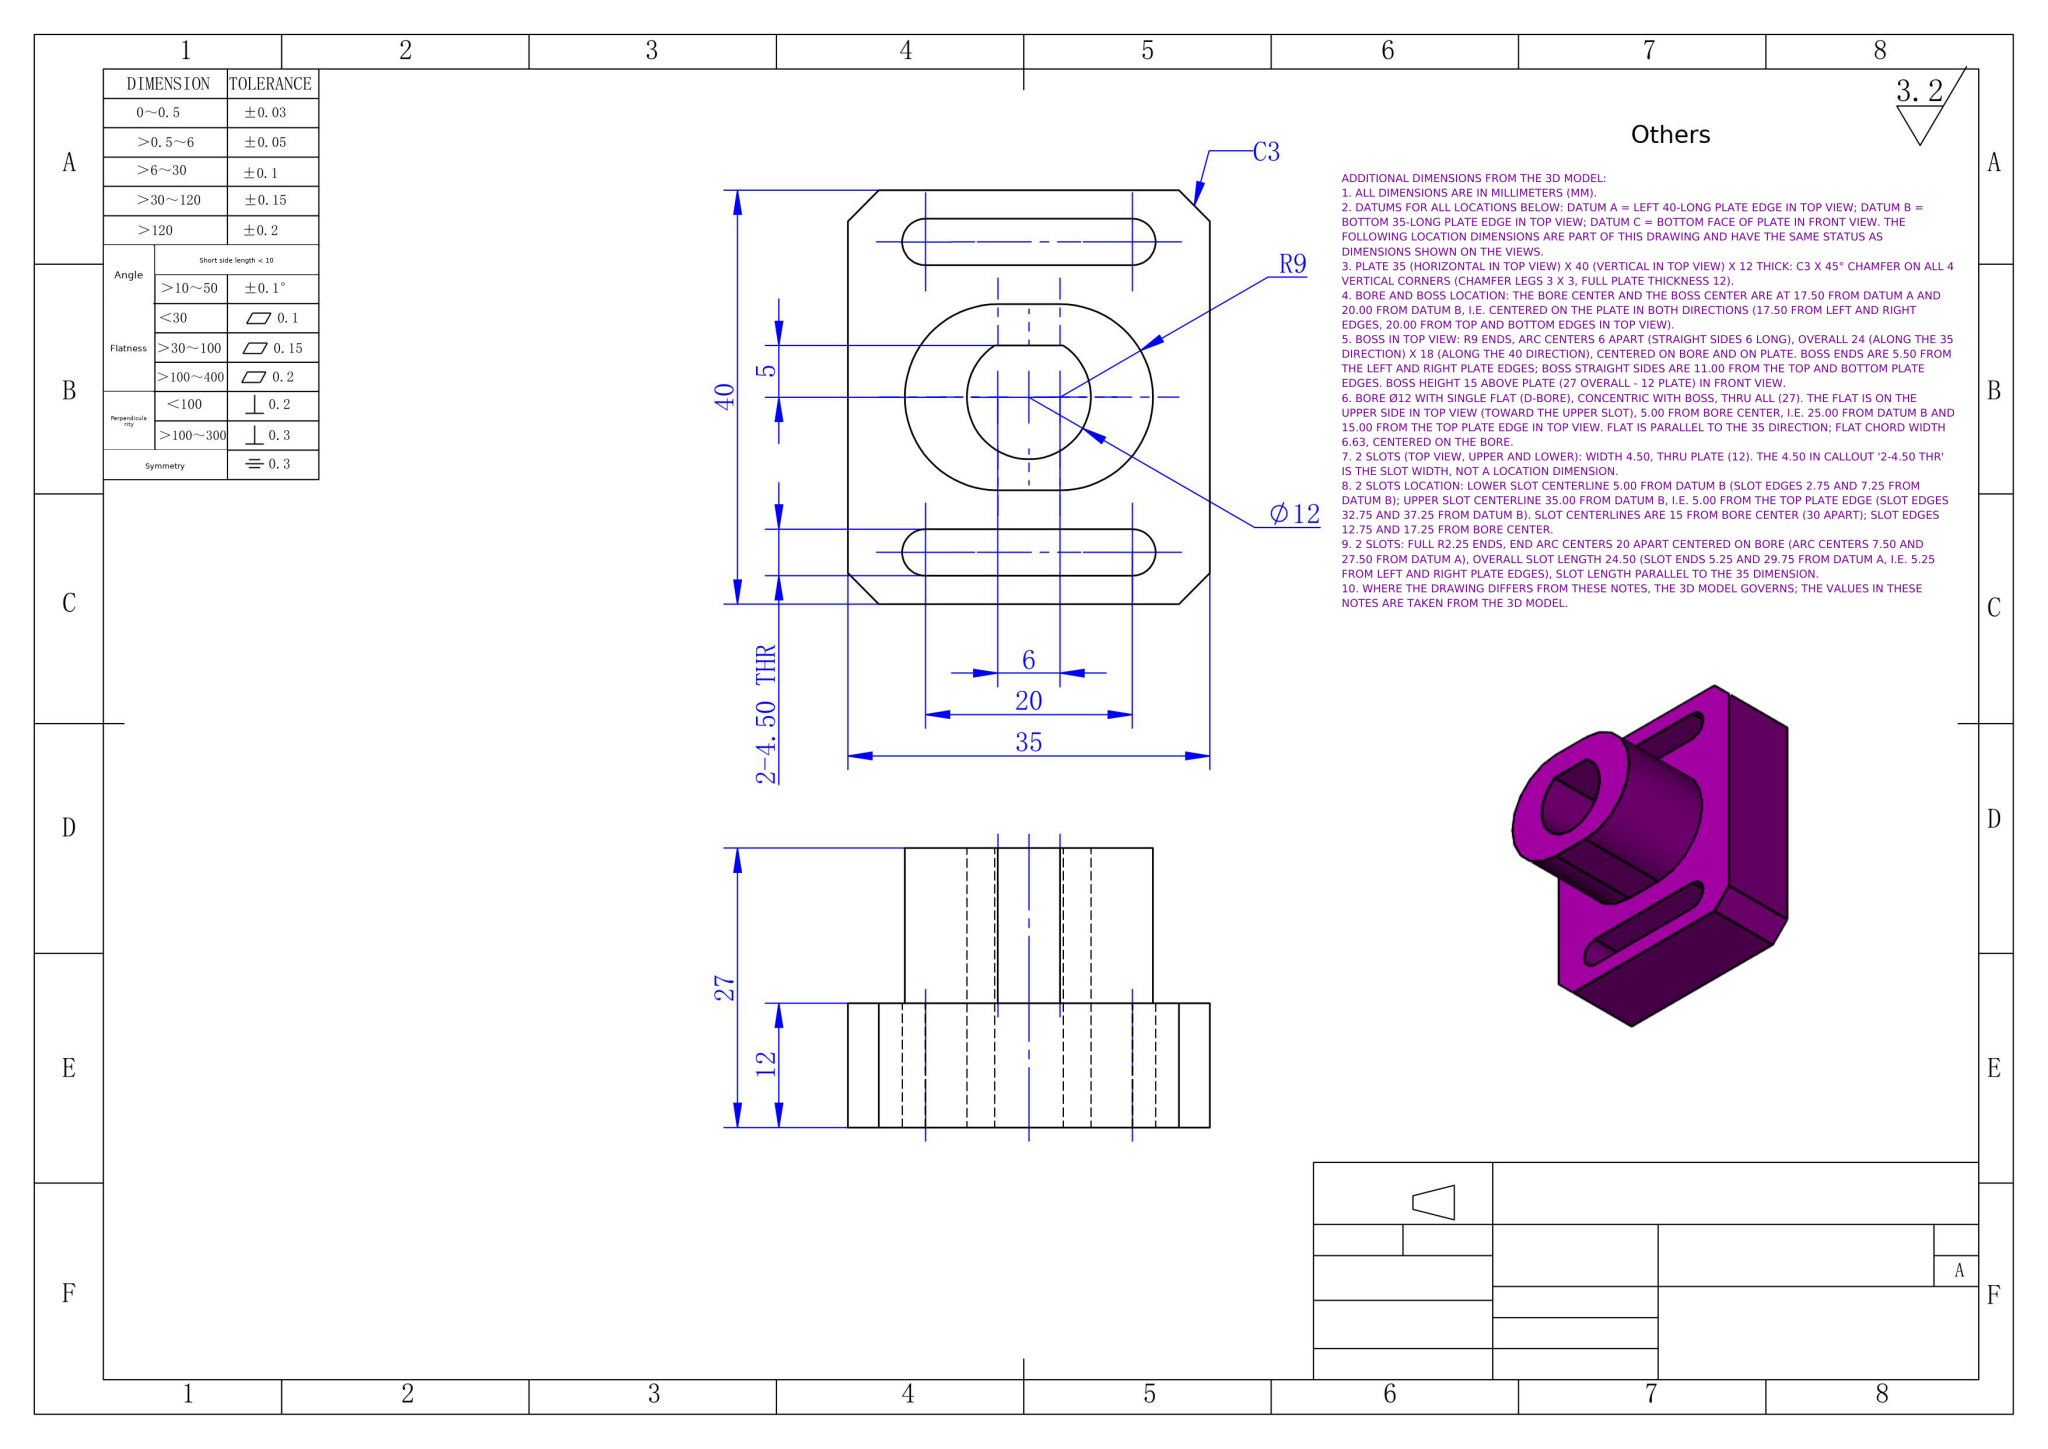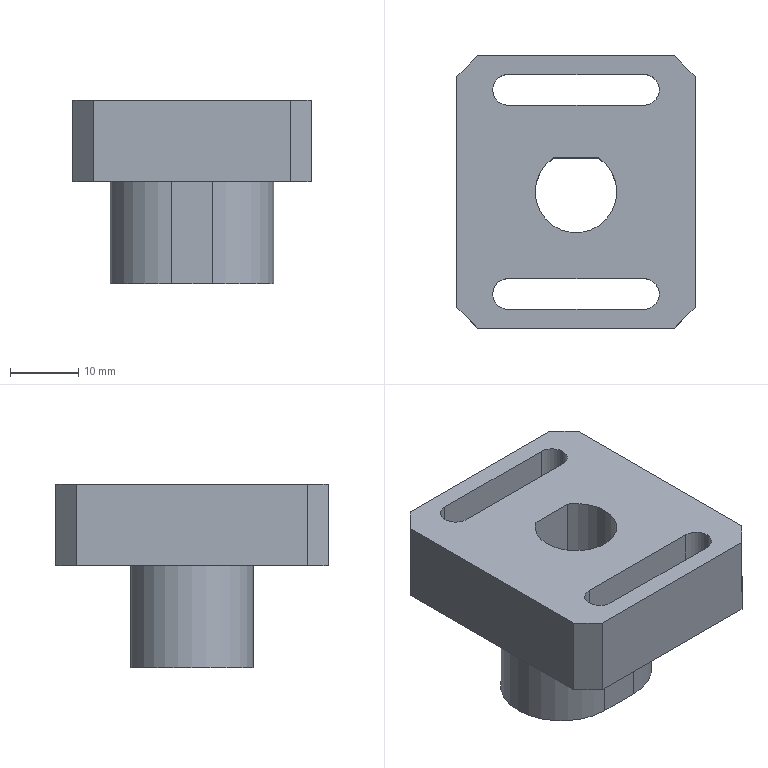Part | NX | mm | 1 solid | 30 faces | box 35 x 40 x 27 mm | volume 16547 mm3 | plane 18 | cylinder 12 | commonest cylinder face diameters 4.5 x6 12 x3 18 x3
STEP:
#1=COLOUR_RGB('',1.,0.,1.);
#2=FILL_AREA_STYLE_COLOUR('',#1);
#3=FILL_AREA_STYLE('',(#2));
#4=SURFACE_STYLE_FILL_AREA(#3);
#5=SURFACE_SIDE_STYLE('',(#4));
#6=SURFACE_STYLE_USAGE(.BOTH.,#5);
#7=PRESENTATION_STYLE_ASSIGNMENT((#6));
#8=CARTESIAN_POINT('',(12.25,-15.,0.));
#9=VERTEX_POINT('',#8);
#10=CARTESIAN_POINT('',(10.,-12.75,0.));
#11=VERTEX_POINT('',#10);
#12=CARTESIAN_POINT('',(10.,-15.,0.));
#13=DIRECTION('',(0.,0.,1.));
#14=DIRECTION('',(1.,0.,0.));
#15=AXIS2_PLACEMENT_3D('',#12,#13,#14);
#16=CIRCLE('',#15,2.25);
#17=EDGE_CURVE('',#9,#11,#16,.T.);
#18=ORIENTED_EDGE('',*,*,#17,.F.);
#19=CARTESIAN_POINT('',(12.25,-15.,12.));
#20=VERTEX_POINT('',#19);
#21=CARTESIAN_POINT('',(12.25,-15.,-15.));
#22=DIRECTION('',(0.,0.,1.));
#23=VECTOR('',#22,1000.);
#24=LINE('',#21,#23);
#25=EDGE_CURVE('',#9,#20,#24,.T.);
#26=ORIENTED_EDGE('',*,*,#25,.T.);
#27=CARTESIAN_POINT('',(10.,-12.75,12.));
#28=VERTEX_POINT('',#27);
#29=CARTESIAN_POINT('',(10.,-15.,12.));
#30=DIRECTION('',(0.,0.,1.));
#31=DIRECTION('',(1.,0.,0.));
#32=AXIS2_PLACEMENT_3D('',#29,#30,#31);
#33=CIRCLE('',#32,2.25);
#34=EDGE_CURVE('',#20,#28,#33,.T.);
#35=ORIENTED_EDGE('',*,*,#34,.T.);
#36=CARTESIAN_POINT('',(10.,-12.75,-15.));
#37=DIRECTION('',(0.,0.,1.));
#38=VECTOR('',#37,1000.);
#39=LINE('',#36,#38);
#40=EDGE_CURVE('',#11,#28,#39,.T.);
#41=ORIENTED_EDGE('',*,*,#40,.F.);
#42=EDGE_LOOP('',(#18,#26,#35,#41));
#43=FACE_OUTER_BOUND('',#42,.T.);
#44=CARTESIAN_POINT('',(10.,-15.,-15.));
#45=DIRECTION('',(0.,0.,1.));
#46=DIRECTION('',(1.,0.,0.));
#47=AXIS2_PLACEMENT_3D('',#44,#45,#46);
#48=CYLINDRICAL_SURFACE('',#47,2.25);
#49=ADVANCED_FACE('',(#43),#48,.F.);
#50=CARTESIAN_POINT('',(12.25,15.,0.));
#51=VERTEX_POINT('',#50);
#52=CARTESIAN_POINT('',(10.,17.25,0.));
#53=VERTEX_POINT('',#52);
#54=CARTESIAN_POINT('',(10.,15.,0.));
#55=DIRECTION('',(0.,0.,1.));
#56=DIRECTION('',(1.,0.,0.));
#57=AXIS2_PLACEMENT_3D('',#54,#55,#56);
#58=CIRCLE('',#57,2.25);
#59=EDGE_CURVE('',#51,#53,#58,.T.);
#60=ORIENTED_EDGE('',*,*,#59,.F.);
#61=CARTESIAN_POINT('',(12.25,15.,12.));
#62=VERTEX_POINT('',#61);
#63=CARTESIAN_POINT('',(12.25,15.,-15.));
#64=DIRECTION('',(0.,0.,1.));
#65=VECTOR('',#64,1000.);
#66=LINE('',#63,#65);
#67=EDGE_CURVE('',#51,#62,#66,.T.);
#68=ORIENTED_EDGE('',*,*,#67,.T.);
#69=CARTESIAN_POINT('',(10.,17.25,12.));
#70=VERTEX_POINT('',#69);
#71=CARTESIAN_POINT('',(10.,15.,12.));
#72=DIRECTION('',(0.,0.,1.));
#73=DIRECTION('',(1.,0.,0.));
#74=AXIS2_PLACEMENT_3D('',#71,#72,#73);
#75=CIRCLE('',#74,2.25);
#76=EDGE_CURVE('',#62,#70,#75,.T.);
#77=ORIENTED_EDGE('',*,*,#76,.T.);
#78=CARTESIAN_POINT('',(10.,17.25,-15.));
#79=DIRECTION('',(0.,0.,1.));
#80=VECTOR('',#79,1000.);
#81=LINE('',#78,#80);
#82=EDGE_CURVE('',#53,#70,#81,.T.);
#83=ORIENTED_EDGE('',*,*,#82,.F.);
#84=EDGE_LOOP('',(#60,#68,#77,#83));
#85=FACE_OUTER_BOUND('',#84,.T.);
#86=CARTESIAN_POINT('',(10.,15.,-15.));
#87=DIRECTION('',(0.,0.,1.));
#88=DIRECTION('',(1.,0.,0.));
#89=AXIS2_PLACEMENT_3D('',#86,#87,#88);
#90=CYLINDRICAL_SURFACE('',#89,2.25);
#91=ADVANCED_FACE('',(#85),#90,.F.);
#92=CARTESIAN_POINT('',(6.,0.,12.));
#93=VERTEX_POINT('',#92);
#94=CARTESIAN_POINT('',(-6.,0.,12.));
#95=VERTEX_POINT('',#94);
#96=CARTESIAN_POINT('',(0.,0.,12.));
#97=DIRECTION('',(0.,0.,-1.));
#98=DIRECTION('',(-1.,0.,0.));
#99=AXIS2_PLACEMENT_3D('',#96,#97,#98);
#100=CIRCLE('',#99,6.);
#101=EDGE_CURVE('',#93,#95,#100,.T.);
#102=ORIENTED_EDGE('',*,*,#101,.F.);
#103=CARTESIAN_POINT('',(6.,0.,-15.));
#104=VERTEX_POINT('',#103);
#105=CARTESIAN_POINT('',(6.,0.,12.));
#106=DIRECTION('',(0.,0.,-1.));
#107=VECTOR('',#106,1000.);
#108=LINE('',#105,#107);
#109=EDGE_CURVE('',#93,#104,#108,.T.);
#110=ORIENTED_EDGE('',*,*,#109,.T.);
#111=CARTESIAN_POINT('',(-6.,0.,-15.));
#112=VERTEX_POINT('',#111);
#113=CARTESIAN_POINT('',(0.,0.,-15.));
#114=DIRECTION('',(0.,0.,-1.));
#115=DIRECTION('',(-1.,0.,0.));
#116=AXIS2_PLACEMENT_3D('',#113,#114,#115);
#117=CIRCLE('',#116,6.);
#118=EDGE_CURVE('',#104,#112,#117,.T.);
#119=ORIENTED_EDGE('',*,*,#118,.T.);
#120=CARTESIAN_POINT('',(-6.,0.,12.));
#121=DIRECTION('',(0.,0.,-1.));
#122=VECTOR('',#121,1000.);
#123=LINE('',#120,#122);
#124=EDGE_CURVE('',#95,#112,#123,.T.);
#125=ORIENTED_EDGE('',*,*,#124,.F.);
#126=EDGE_LOOP('',(#102,#110,#119,#125));
#127=FACE_OUTER_BOUND('',#126,.T.);
#128=CARTESIAN_POINT('',(0.,0.,12.));
#129=DIRECTION('',(0.,0.,-1.));
#130=DIRECTION('',(-1.,0.,0.));
#131=AXIS2_PLACEMENT_3D('',#128,#129,#130);
#132=CYLINDRICAL_SURFACE('',#131,6.);
#133=ADVANCED_FACE('',(#127),#132,.F.);
#134=CARTESIAN_POINT('',(-3.317,5.,12.));
#135=VERTEX_POINT('',#134);
#136=CARTESIAN_POINT('',(0.,0.,12.));
#137=DIRECTION('',(0.,0.,-1.));
#138=DIRECTION('',(-1.,0.,0.));
#139=AXIS2_PLACEMENT_3D('',#136,#137,#138);
#140=CIRCLE('',#139,6.);
#141=EDGE_CURVE('',#95,#135,#140,.T.);
#142=ORIENTED_EDGE('',*,*,#141,.F.);
#143=ORIENTED_EDGE('',*,*,#124,.T.);
#144=CARTESIAN_POINT('',(-3.317,5.,-15.));
#145=VERTEX_POINT('',#144);
#146=CARTESIAN_POINT('',(0.,0.,-15.));
#147=DIRECTION('',(0.,0.,-1.));
#148=DIRECTION('',(-1.,0.,0.));
#149=AXIS2_PLACEMENT_3D('',#146,#147,#148);
#150=CIRCLE('',#149,6.);
#151=EDGE_CURVE('',#112,#145,#150,.T.);
#152=ORIENTED_EDGE('',*,*,#151,.T.);
#153=CARTESIAN_POINT('',(-3.317,5.,12.));
#154=DIRECTION('',(0.,0.,-1.));
#155=VECTOR('',#154,1000.);
#156=LINE('',#153,#155);
#157=EDGE_CURVE('',#135,#145,#156,.T.);
#158=ORIENTED_EDGE('',*,*,#157,.F.);
#159=EDGE_LOOP('',(#142,#143,#152,#158));
#160=FACE_OUTER_BOUND('',#159,.T.);
#161=CARTESIAN_POINT('',(0.,0.,12.));
#162=DIRECTION('',(0.,0.,-1.));
#163=DIRECTION('',(-1.,0.,0.));
#164=AXIS2_PLACEMENT_3D('',#161,#162,#163);
#165=CYLINDRICAL_SURFACE('',#164,6.);
#166=ADVANCED_FACE('',(#160),#165,.F.);
#167=CARTESIAN_POINT('',(12.,0.,-15.));
#168=VERTEX_POINT('',#167);
#169=CARTESIAN_POINT('',(3.,-9.,-15.));
#170=VERTEX_POINT('',#169);
#171=CARTESIAN_POINT('',(3.,0.,-15.));
#172=DIRECTION('',(0.,0.,-1.));
#173=DIRECTION('',(-1.,0.,0.));
#174=AXIS2_PLACEMENT_3D('',#171,#172,#173);
#175=CIRCLE('',#174,9.);
#176=EDGE_CURVE('',#168,#170,#175,.T.);
#177=ORIENTED_EDGE('',*,*,#176,.F.);
#178=CARTESIAN_POINT('',(12.,0.,0.));
#179=VERTEX_POINT('',#178);
#180=CARTESIAN_POINT('',(12.,0.,-15.));
#181=DIRECTION('',(0.,0.,1.));
#182=VECTOR('',#181,1000.);
#183=LINE('',#180,#182);
#184=EDGE_CURVE('',#168,#179,#183,.T.);
#185=ORIENTED_EDGE('',*,*,#184,.T.);
#186=CARTESIAN_POINT('',(3.,-9.,0.));
#187=VERTEX_POINT('',#186);
#188=CARTESIAN_POINT('',(3.,0.,0.));
#189=DIRECTION('',(0.,0.,-1.));
#190=DIRECTION('',(-1.,0.,0.));
#191=AXIS2_PLACEMENT_3D('',#188,#189,#190);
#192=CIRCLE('',#191,9.);
#193=EDGE_CURVE('',#179,#187,#192,.T.);
#194=ORIENTED_EDGE('',*,*,#193,.T.);
#195=CARTESIAN_POINT('',(3.,-9.,-15.));
#196=DIRECTION('',(0.,0.,1.));
#197=VECTOR('',#196,1000.);
#198=LINE('',#195,#197);
#199=EDGE_CURVE('',#170,#187,#198,.T.);
#200=ORIENTED_EDGE('',*,*,#199,.F.);
#201=EDGE_LOOP('',(#177,#185,#194,#200));
#202=FACE_OUTER_BOUND('',#201,.T.);
#203=CARTESIAN_POINT('',(3.,0.,-15.));
#204=DIRECTION('',(0.,0.,1.));
#205=DIRECTION('',(1.,0.,0.));
#206=AXIS2_PLACEMENT_3D('',#203,#204,#205);
#207=CYLINDRICAL_SURFACE('',#206,9.);
#208=ADVANCED_FACE('',(#202),#207,.T.);
#209=CARTESIAN_POINT('',(-10.,-12.75,0.));
#210=VERTEX_POINT('',#209);
#211=CARTESIAN_POINT('',(0.,-12.75,0.));
#212=DIRECTION('',(-1.,0.,0.));
#213=VECTOR('',#212,1000.);
#214=LINE('',#211,#213);
#215=EDGE_CURVE('',#11,#210,#214,.T.);
#216=ORIENTED_EDGE('',*,*,#215,.T.);
#217=CARTESIAN_POINT('',(-10.,-17.25,0.));
#218=VERTEX_POINT('',#217);
#219=CARTESIAN_POINT('',(-10.,-15.,0.));
#220=DIRECTION('',(0.,0.,1.));
#221=DIRECTION('',(1.,0.,0.));
#222=AXIS2_PLACEMENT_3D('',#219,#220,#221);
#223=CIRCLE('',#222,2.25);
#224=EDGE_CURVE('',#210,#218,#223,.T.);
#225=ORIENTED_EDGE('',*,*,#224,.T.);
#226=CARTESIAN_POINT('',(10.,-17.25,0.));
#227=VERTEX_POINT('',#226);
#228=CARTESIAN_POINT('',(0.,-17.25,0.));
#229=DIRECTION('',(1.,0.,0.));
#230=VECTOR('',#229,1000.);
#231=LINE('',#228,#230);
#232=EDGE_CURVE('',#218,#227,#231,.T.);
#233=ORIENTED_EDGE('',*,*,#232,.T.);
#234=CARTESIAN_POINT('',(10.,-15.,0.));
#235=DIRECTION('',(0.,0.,1.));
#236=DIRECTION('',(1.,0.,0.));
#237=AXIS2_PLACEMENT_3D('',#234,#235,#236);
#238=CIRCLE('',#237,2.25);
#239=EDGE_CURVE('',#227,#9,#238,.T.);
#240=ORIENTED_EDGE('',*,*,#239,.T.);
#241=ORIENTED_EDGE('',*,*,#17,.T.);
#242=EDGE_LOOP('',(#216,#225,#233,#240,#241));
#243=FACE_BOUND('',#242,.T.);
#244=CARTESIAN_POINT('',(-10.,17.25,0.));
#245=VERTEX_POINT('',#244);
#246=CARTESIAN_POINT('',(0.,17.25,0.));
#247=DIRECTION('',(-1.,0.,0.));
#248=VECTOR('',#247,1000.);
#249=LINE('',#246,#248);
#250=EDGE_CURVE('',#53,#245,#249,.T.);
#251=ORIENTED_EDGE('',*,*,#250,.T.);
#252=CARTESIAN_POINT('',(-10.,12.75,0.));
#253=VERTEX_POINT('',#252);
#254=CARTESIAN_POINT('',(-10.,15.,0.));
#255=DIRECTION('',(0.,0.,1.));
#256=DIRECTION('',(1.,0.,0.));
#257=AXIS2_PLACEMENT_3D('',#254,#255,#256);
#258=CIRCLE('',#257,2.25);
#259=EDGE_CURVE('',#245,#253,#258,.T.);
#260=ORIENTED_EDGE('',*,*,#259,.T.);
#261=CARTESIAN_POINT('',(10.,12.75,0.));
#262=VERTEX_POINT('',#261);
#263=CARTESIAN_POINT('',(0.,12.75,0.));
#264=DIRECTION('',(1.,0.,0.));
#265=VECTOR('',#264,1000.);
#266=LINE('',#263,#265);
#267=EDGE_CURVE('',#253,#262,#266,.T.);
#268=ORIENTED_EDGE('',*,*,#267,.T.);
#269=CARTESIAN_POINT('',(10.,15.,0.));
#270=DIRECTION('',(0.,0.,1.));
#271=DIRECTION('',(1.,0.,0.));
#272=AXIS2_PLACEMENT_3D('',#269,#270,#271);
#273=CIRCLE('',#272,2.25);
#274=EDGE_CURVE('',#262,#51,#273,.T.);
#275=ORIENTED_EDGE('',*,*,#274,.T.);
#276=ORIENTED_EDGE('',*,*,#59,.T.);
#277=EDGE_LOOP('',(#251,#260,#268,#275,#276));
#278=FACE_BOUND('',#277,.T.);
#279=CARTESIAN_POINT('',(17.5,-17.,0.));
#280=VERTEX_POINT('',#279);
#281=CARTESIAN_POINT('',(17.5,17.,0.));
#282=VERTEX_POINT('',#281);
#283=CARTESIAN_POINT('',(17.5,20.,0.));
#284=DIRECTION('',(-0.,1.,0.));
#285=VECTOR('',#284,1000.);
#286=LINE('',#283,#285);
#287=EDGE_CURVE('',#280,#282,#286,.T.);
#288=ORIENTED_EDGE('',*,*,#287,.F.);
#289=CARTESIAN_POINT('',(14.5,-20.,0.));
#290=VERTEX_POINT('',#289);
#291=CARTESIAN_POINT('',(17.5,-17.,0.));
#292=DIRECTION('',(-0.7071,-0.7071,0.));
#293=VECTOR('',#292,1000.);
#294=LINE('',#291,#293);
#295=EDGE_CURVE('',#280,#290,#294,.T.);
#296=ORIENTED_EDGE('',*,*,#295,.T.);
#297=CARTESIAN_POINT('',(-14.5,-20.,0.));
#298=VERTEX_POINT('',#297);
#299=CARTESIAN_POINT('',(-17.5,-20.,0.));
#300=DIRECTION('',(1.,0.,0.));
#301=VECTOR('',#300,1000.);
#302=LINE('',#299,#301);
#303=EDGE_CURVE('',#298,#290,#302,.T.);
#304=ORIENTED_EDGE('',*,*,#303,.F.);
#305=CARTESIAN_POINT('',(-17.5,-17.,0.));
#306=VERTEX_POINT('',#305);
#307=CARTESIAN_POINT('',(-14.5,-20.,0.));
#308=DIRECTION('',(-0.7071,0.7071,0.));
#309=VECTOR('',#308,1000.);
#310=LINE('',#307,#309);
#311=EDGE_CURVE('',#298,#306,#310,.T.);
#312=ORIENTED_EDGE('',*,*,#311,.T.);
#313=CARTESIAN_POINT('',(-17.5,17.,0.));
#314=VERTEX_POINT('',#313);
#315=CARTESIAN_POINT('',(-17.5,20.,0.));
#316=DIRECTION('',(0.,-1.,0.));
#317=VECTOR('',#316,1000.);
#318=LINE('',#315,#317);
#319=EDGE_CURVE('',#314,#306,#318,.T.);
#320=ORIENTED_EDGE('',*,*,#319,.F.);
#321=CARTESIAN_POINT('',(-14.5,20.,0.));
#322=VERTEX_POINT('',#321);
#323=CARTESIAN_POINT('',(-17.5,17.,0.));
#324=DIRECTION('',(0.7071,0.7071,0.));
#325=VECTOR('',#324,1000.);
#326=LINE('',#323,#325);
#327=EDGE_CURVE('',#314,#322,#326,.T.);
#328=ORIENTED_EDGE('',*,*,#327,.T.);
#329=CARTESIAN_POINT('',(14.5,20.,0.));
#330=VERTEX_POINT('',#329);
#331=CARTESIAN_POINT('',(-17.5,20.,0.));
#332=DIRECTION('',(-1.,0.,0.));
#333=VECTOR('',#332,1000.);
#334=LINE('',#331,#333);
#335=EDGE_CURVE('',#330,#322,#334,.T.);
#336=ORIENTED_EDGE('',*,*,#335,.F.);
#337=CARTESIAN_POINT('',(14.5,20.,0.));
#338=DIRECTION('',(0.7071,-0.7071,0.));
#339=VECTOR('',#338,1000.);
#340=LINE('',#337,#339);
#341=EDGE_CURVE('',#330,#282,#340,.T.);
#342=ORIENTED_EDGE('',*,*,#341,.T.);
#343=EDGE_LOOP('',(#288,#296,#304,#312,#320,#328,#336,#342));
#344=FACE_OUTER_BOUND('',#343,.T.);
#345=CARTESIAN_POINT('',(3.,9.,0.));
#346=VERTEX_POINT('',#345);
#347=CARTESIAN_POINT('',(3.,0.,0.));
#348=DIRECTION('',(0.,0.,-1.));
#349=DIRECTION('',(-1.,0.,0.));
#350=AXIS2_PLACEMENT_3D('',#347,#348,#349);
#351=CIRCLE('',#350,9.);
#352=EDGE_CURVE('',#346,#179,#351,.T.);
#353=ORIENTED_EDGE('',*,*,#352,.F.);
#354=CARTESIAN_POINT('',(-3.,9.,0.));
#355=VERTEX_POINT('',#354);
#356=CARTESIAN_POINT('',(3.,9.,0.));
#357=DIRECTION('',(1.,-0.,0.));
#358=VECTOR('',#357,1000.);
#359=LINE('',#356,#358);
#360=EDGE_CURVE('',#355,#346,#359,.T.);
#361=ORIENTED_EDGE('',*,*,#360,.F.);
#362=CARTESIAN_POINT('',(-3.,-9.,0.));
#363=VERTEX_POINT('',#362);
#364=CARTESIAN_POINT('',(-3.,0.,0.));
#365=DIRECTION('',(0.,0.,-1.));
#366=DIRECTION('',(-1.,0.,0.));
#367=AXIS2_PLACEMENT_3D('',#364,#365,#366);
#368=CIRCLE('',#367,9.);
#369=EDGE_CURVE('',#363,#355,#368,.T.);
#370=ORIENTED_EDGE('',*,*,#369,.F.);
#371=CARTESIAN_POINT('',(3.,-9.,0.));
#372=DIRECTION('',(-1.,0.,0.));
#373=VECTOR('',#372,1000.);
#374=LINE('',#371,#373);
#375=EDGE_CURVE('',#187,#363,#374,.T.);
#376=ORIENTED_EDGE('',*,*,#375,.F.);
#377=ORIENTED_EDGE('',*,*,#193,.F.);
#378=EDGE_LOOP('',(#353,#361,#370,#376,#377));
#379=FACE_BOUND('',#378,.T.);
#380=CARTESIAN_POINT('',(0.,0.,0.));
#381=DIRECTION('',(0.,0.,1.));
#382=DIRECTION('',(1.,0.,0.));
#383=AXIS2_PLACEMENT_3D('',#380,#381,#382);
#384=PLANE('',#383);
#385=ADVANCED_FACE('',(#243,#278,#344,#379),#384,.F.);
#386=CARTESIAN_POINT('',(17.5,-17.,12.));
#387=VERTEX_POINT('',#386);
#388=CARTESIAN_POINT('',(17.5,17.,12.));
#389=VERTEX_POINT('',#388);
#390=CARTESIAN_POINT('',(17.5,20.,12.));
#391=DIRECTION('',(-0.,1.,0.));
#392=VECTOR('',#391,1000.);
#393=LINE('',#390,#392);
#394=EDGE_CURVE('',#387,#389,#393,.T.);
#395=ORIENTED_EDGE('',*,*,#394,.F.);
#396=CARTESIAN_POINT('',(17.5,-17.,12.));
#397=DIRECTION('',(0.,0.,-1.));
#398=VECTOR('',#397,1000.);
#399=LINE('',#396,#398);
#400=EDGE_CURVE('',#387,#280,#399,.T.);
#401=ORIENTED_EDGE('',*,*,#400,.T.);
#402=ORIENTED_EDGE('',*,*,#287,.T.);
#403=CARTESIAN_POINT('',(17.5,17.,12.));
#404=DIRECTION('',(0.,0.,1.));
#405=VECTOR('',#404,1000.);
#406=LINE('',#403,#405);
#407=EDGE_CURVE('',#282,#389,#406,.T.);
#408=ORIENTED_EDGE('',*,*,#407,.T.);
#409=EDGE_LOOP('',(#395,#401,#402,#408));
#410=FACE_OUTER_BOUND('',#409,.T.);
#411=CARTESIAN_POINT('',(17.5,20.,12.));
#412=DIRECTION('',(-1.,-0.,0.));
#413=DIRECTION('',(0.,-1.,0.));
#414=AXIS2_PLACEMENT_3D('',#411,#412,#413);
#415=PLANE('',#414);
#416=ADVANCED_FACE('',(#410),#415,.F.);
#417=ORIENTED_EDGE('',*,*,#335,.T.);
#418=CARTESIAN_POINT('',(-14.5,20.,12.));
#419=VERTEX_POINT('',#418);
#420=CARTESIAN_POINT('',(-14.5,20.,12.));
#421=DIRECTION('',(0.,0.,1.));
#422=VECTOR('',#421,1000.);
#423=LINE('',#420,#422);
#424=EDGE_CURVE('',#322,#419,#423,.T.);
#425=ORIENTED_EDGE('',*,*,#424,.T.);
#426=CARTESIAN_POINT('',(14.5,20.,12.));
#427=VERTEX_POINT('',#426);
#428=CARTESIAN_POINT('',(-17.5,20.,12.));
#429=DIRECTION('',(-1.,0.,0.));
#430=VECTOR('',#429,1000.);
#431=LINE('',#428,#430);
#432=EDGE_CURVE('',#427,#419,#431,.T.);
#433=ORIENTED_EDGE('',*,*,#432,.F.);
#434=CARTESIAN_POINT('',(14.5,20.,12.));
#435=DIRECTION('',(0.,0.,-1.));
#436=VECTOR('',#435,1000.);
#437=LINE('',#434,#436);
#438=EDGE_CURVE('',#427,#330,#437,.T.);
#439=ORIENTED_EDGE('',*,*,#438,.T.);
#440=EDGE_LOOP('',(#417,#425,#433,#439));
#441=FACE_OUTER_BOUND('',#440,.T.);
#442=CARTESIAN_POINT('',(-17.5,20.,12.));
#443=DIRECTION('',(0.,-1.,0.));
#444=DIRECTION('',(0.,0.,-1.));
#445=AXIS2_PLACEMENT_3D('',#442,#443,#444);
#446=PLANE('',#445);
#447=ADVANCED_FACE('',(#441),#446,.F.);
#448=ORIENTED_EDGE('',*,*,#319,.T.);
#449=CARTESIAN_POINT('',(-17.5,-17.,12.));
#450=VERTEX_POINT('',#449);
#451=CARTESIAN_POINT('',(-17.5,-17.,12.));
#452=DIRECTION('',(0.,0.,1.));
#453=VECTOR('',#452,1000.);
#454=LINE('',#451,#453);
#455=EDGE_CURVE('',#306,#450,#454,.T.);
#456=ORIENTED_EDGE('',*,*,#455,.T.);
#457=CARTESIAN_POINT('',(-17.5,17.,12.));
#458=VERTEX_POINT('',#457);
#459=CARTESIAN_POINT('',(-17.5,20.,12.));
#460=DIRECTION('',(0.,-1.,0.));
#461=VECTOR('',#460,1000.);
#462=LINE('',#459,#461);
#463=EDGE_CURVE('',#458,#450,#462,.T.);
#464=ORIENTED_EDGE('',*,*,#463,.F.);
#465=CARTESIAN_POINT('',(-17.5,17.,12.));
#466=DIRECTION('',(0.,0.,-1.));
#467=VECTOR('',#466,1000.);
#468=LINE('',#465,#467);
#469=EDGE_CURVE('',#458,#314,#468,.T.);
#470=ORIENTED_EDGE('',*,*,#469,.T.);
#471=EDGE_LOOP('',(#448,#456,#464,#470));
#472=FACE_OUTER_BOUND('',#471,.T.);
#473=CARTESIAN_POINT('',(-17.5,20.,12.));
#474=DIRECTION('',(1.,0.,0.));
#475=DIRECTION('',(-0.,1.,0.));
#476=AXIS2_PLACEMENT_3D('',#473,#474,#475);
#477=PLANE('',#476);
#478=ADVANCED_FACE('',(#472),#477,.F.);
#479=ORIENTED_EDGE('',*,*,#303,.T.);
#480=CARTESIAN_POINT('',(14.5,-20.,12.));
#481=VERTEX_POINT('',#480);
#482=CARTESIAN_POINT('',(14.5,-20.,12.));
#483=DIRECTION('',(0.,0.,1.));
#484=VECTOR('',#483,1000.);
#485=LINE('',#482,#484);
#486=EDGE_CURVE('',#290,#481,#485,.T.);
#487=ORIENTED_EDGE('',*,*,#486,.T.);
#488=CARTESIAN_POINT('',(-14.5,-20.,12.));
#489=VERTEX_POINT('',#488);
#490=CARTESIAN_POINT('',(-17.5,-20.,12.));
#491=DIRECTION('',(1.,0.,0.));
#492=VECTOR('',#491,1000.);
#493=LINE('',#490,#492);
#494=EDGE_CURVE('',#489,#481,#493,.T.);
#495=ORIENTED_EDGE('',*,*,#494,.F.);
#496=CARTESIAN_POINT('',(-14.5,-20.,12.));
#497=DIRECTION('',(0.,0.,-1.));
#498=VECTOR('',#497,1000.);
#499=LINE('',#496,#498);
#500=EDGE_CURVE('',#489,#298,#499,.T.);
#501=ORIENTED_EDGE('',*,*,#500,.T.);
#502=EDGE_LOOP('',(#479,#487,#495,#501));
#503=FACE_OUTER_BOUND('',#502,.T.);
#504=CARTESIAN_POINT('',(-17.5,-20.,12.));
#505=DIRECTION('',(0.,1.,0.));
#506=DIRECTION('',(0.,0.,1.));
#507=AXIS2_PLACEMENT_3D('',#504,#505,#506);
#508=PLANE('',#507);
#509=ADVANCED_FACE('',(#503),#508,.F.);
#510=CARTESIAN_POINT('',(-10.,-12.75,12.));
#511=VERTEX_POINT('',#510);
#512=CARTESIAN_POINT('',(-10.,-17.25,12.));
#513=VERTEX_POINT('',#512);
#514=CARTESIAN_POINT('',(-10.,-15.,12.));
#515=DIRECTION('',(0.,0.,1.));
#516=DIRECTION('',(1.,0.,0.));
#517=AXIS2_PLACEMENT_3D('',#514,#515,#516);
#518=CIRCLE('',#517,2.25);
#519=EDGE_CURVE('',#511,#513,#518,.T.);
#520=ORIENTED_EDGE('',*,*,#519,.F.);
#521=CARTESIAN_POINT('',(-10.,-12.75,12.));
#522=DIRECTION('',(-1.,0.,0.));
#523=VECTOR('',#522,1000.);
#524=LINE('',#521,#523);
#525=EDGE_CURVE('',#28,#511,#524,.T.);
#526=ORIENTED_EDGE('',*,*,#525,.F.);
#527=ORIENTED_EDGE('',*,*,#34,.F.);
#528=CARTESIAN_POINT('',(10.,-17.25,12.));
#529=VERTEX_POINT('',#528);
#530=CARTESIAN_POINT('',(10.,-15.,12.));
#531=DIRECTION('',(0.,0.,1.));
#532=DIRECTION('',(1.,0.,0.));
#533=AXIS2_PLACEMENT_3D('',#530,#531,#532);
#534=CIRCLE('',#533,2.25);
#535=EDGE_CURVE('',#529,#20,#534,.T.);
#536=ORIENTED_EDGE('',*,*,#535,.F.);
#537=CARTESIAN_POINT('',(-10.,-17.25,12.));
#538=DIRECTION('',(1.,0.,0.));
#539=VECTOR('',#538,1000.);
#540=LINE('',#537,#539);
#541=EDGE_CURVE('',#513,#529,#540,.T.);
#542=ORIENTED_EDGE('',*,*,#541,.F.);
#543=EDGE_LOOP('',(#520,#526,#527,#536,#542));
#544=FACE_BOUND('',#543,.T.);
#545=CARTESIAN_POINT('',(-10.,17.25,12.));
#546=VERTEX_POINT('',#545);
#547=CARTESIAN_POINT('',(-10.,12.75,12.));
#548=VERTEX_POINT('',#547);
#549=CARTESIAN_POINT('',(-10.,15.,12.));
#550=DIRECTION('',(0.,0.,1.));
#551=DIRECTION('',(1.,0.,0.));
#552=AXIS2_PLACEMENT_3D('',#549,#550,#551);
#553=CIRCLE('',#552,2.25);
#554=EDGE_CURVE('',#546,#548,#553,.T.);
#555=ORIENTED_EDGE('',*,*,#554,.F.);
#556=CARTESIAN_POINT('',(-10.,17.25,12.));
#557=DIRECTION('',(-1.,0.,0.));
#558=VECTOR('',#557,1000.);
#559=LINE('',#556,#558);
#560=EDGE_CURVE('',#70,#546,#559,.T.);
#561=ORIENTED_EDGE('',*,*,#560,.F.);
#562=ORIENTED_EDGE('',*,*,#76,.F.);
#563=CARTESIAN_POINT('',(10.,12.75,12.));
#564=VERTEX_POINT('',#563);
#565=CARTESIAN_POINT('',(10.,15.,12.));
#566=DIRECTION('',(0.,0.,1.));
#567=DIRECTION('',(1.,0.,0.));
#568=AXIS2_PLACEMENT_3D('',#565,#566,#567);
#569=CIRCLE('',#568,2.25);
#570=EDGE_CURVE('',#564,#62,#569,.T.);
#571=ORIENTED_EDGE('',*,*,#570,.F.);
#572=CARTESIAN_POINT('',(-10.,12.75,12.));
#573=DIRECTION('',(1.,0.,0.));
#574=VECTOR('',#573,1000.);
#575=LINE('',#572,#574);
#576=EDGE_CURVE('',#548,#564,#575,.T.);
#577=ORIENTED_EDGE('',*,*,#576,.F.);
#578=EDGE_LOOP('',(#555,#561,#562,#571,#577));
#579=FACE_BOUND('',#578,.T.);
#580=CARTESIAN_POINT('',(3.317,5.,12.));
#581=VERTEX_POINT('',#580);
#582=CARTESIAN_POINT('',(0.,0.,12.));
#583=DIRECTION('',(0.,0.,-1.));
#584=DIRECTION('',(-1.,0.,0.));
#585=AXIS2_PLACEMENT_3D('',#582,#583,#584);
#586=CIRCLE('',#585,6.);
#587=EDGE_CURVE('',#581,#93,#586,.T.);
#588=ORIENTED_EDGE('',*,*,#587,.T.);
#589=ORIENTED_EDGE('',*,*,#101,.T.);
#590=ORIENTED_EDGE('',*,*,#141,.T.);
#591=CARTESIAN_POINT('',(3.317,5.,12.));
#592=DIRECTION('',(1.,0.,0.));
#593=VECTOR('',#592,1000.);
#594=LINE('',#591,#593);
#595=EDGE_CURVE('',#135,#581,#594,.T.);
#596=ORIENTED_EDGE('',*,*,#595,.T.);
#597=EDGE_LOOP('',(#588,#589,#590,#596));
#598=FACE_BOUND('',#597,.T.);
#599=ORIENTED_EDGE('',*,*,#494,.T.);
#600=CARTESIAN_POINT('',(17.25,-17.25,12.));
#601=DIRECTION('',(0.7071,0.7071,0.));
#602=VECTOR('',#601,1000.);
#603=LINE('',#600,#602);
#604=EDGE_CURVE('',#481,#387,#603,.T.);
#605=ORIENTED_EDGE('',*,*,#604,.T.);
#606=ORIENTED_EDGE('',*,*,#394,.T.);
#607=CARTESIAN_POINT('',(17.25,17.25,12.));
#608=DIRECTION('',(-0.7071,0.7071,0.));
#609=VECTOR('',#608,1000.);
#610=LINE('',#607,#609);
#611=EDGE_CURVE('',#389,#427,#610,.T.);
#612=ORIENTED_EDGE('',*,*,#611,.T.);
#613=ORIENTED_EDGE('',*,*,#432,.T.);
#614=CARTESIAN_POINT('',(-17.25,17.25,12.));
#615=DIRECTION('',(-0.7071,-0.7071,0.));
#616=VECTOR('',#615,1000.);
#617=LINE('',#614,#616);
#618=EDGE_CURVE('',#419,#458,#617,.T.);
#619=ORIENTED_EDGE('',*,*,#618,.T.);
#620=ORIENTED_EDGE('',*,*,#463,.T.);
#621=CARTESIAN_POINT('',(-17.25,-17.25,12.));
#622=DIRECTION('',(0.7071,-0.7071,0.));
#623=VECTOR('',#622,1000.);
#624=LINE('',#621,#623);
#625=EDGE_CURVE('',#450,#489,#624,.T.);
#626=ORIENTED_EDGE('',*,*,#625,.T.);
#627=EDGE_LOOP('',(#599,#605,#606,#612,#613,#619,#620,#626));
#628=FACE_OUTER_BOUND('',#627,.T.);
#629=CARTESIAN_POINT('',(0.,0.,12.));
#630=DIRECTION('',(0.,0.,1.));
#631=DIRECTION('',(1.,0.,0.));
#632=AXIS2_PLACEMENT_3D('',#629,#630,#631);
#633=PLANE('',#632);
#634=ADVANCED_FACE('',(#544,#579,#598,#628),#633,.T.);
#635=ORIENTED_EDGE('',*,*,#184,.F.);
#636=CARTESIAN_POINT('',(3.,9.,-15.));
#637=VERTEX_POINT('',#636);
#638=CARTESIAN_POINT('',(3.,0.,-15.));
#639=DIRECTION('',(0.,0.,-1.));
#640=DIRECTION('',(-1.,0.,0.));
#641=AXIS2_PLACEMENT_3D('',#638,#639,#640);
#642=CIRCLE('',#641,9.);
#643=EDGE_CURVE('',#637,#168,#642,.T.);
#644=ORIENTED_EDGE('',*,*,#643,.F.);
#645=CARTESIAN_POINT('',(3.,9.,-15.));
#646=DIRECTION('',(0.,0.,1.));
#647=VECTOR('',#646,1000.);
#648=LINE('',#645,#647);
#649=EDGE_CURVE('',#637,#346,#648,.T.);
#650=ORIENTED_EDGE('',*,*,#649,.T.);
#651=ORIENTED_EDGE('',*,*,#352,.T.);
#652=EDGE_LOOP('',(#635,#644,#650,#651));
#653=FACE_OUTER_BOUND('',#652,.T.);
#654=CARTESIAN_POINT('',(3.,0.,-15.));
#655=DIRECTION('',(0.,0.,1.));
#656=DIRECTION('',(1.,0.,0.));
#657=AXIS2_PLACEMENT_3D('',#654,#655,#656);
#658=CYLINDRICAL_SURFACE('',#657,9.);
#659=ADVANCED_FACE('',(#653),#658,.T.);
#660=ORIENTED_EDGE('',*,*,#375,.T.);
#661=CARTESIAN_POINT('',(-3.,-9.,-15.));
#662=VERTEX_POINT('',#661);
#663=CARTESIAN_POINT('',(-3.,-9.,-15.));
#664=DIRECTION('',(0.,0.,1.));
#665=VECTOR('',#664,1000.);
#666=LINE('',#663,#665);
#667=EDGE_CURVE('',#662,#363,#666,.T.);
#668=ORIENTED_EDGE('',*,*,#667,.F.);
#669=CARTESIAN_POINT('',(3.,-9.,-15.));
#670=DIRECTION('',(-1.,0.,0.));
#671=VECTOR('',#670,1000.);
#672=LINE('',#669,#671);
#673=EDGE_CURVE('',#170,#662,#672,.T.);
#674=ORIENTED_EDGE('',*,*,#673,.F.);
#675=ORIENTED_EDGE('',*,*,#199,.T.);
#676=EDGE_LOOP('',(#660,#668,#674,#675));
#677=FACE_OUTER_BOUND('',#676,.T.);
#678=CARTESIAN_POINT('',(3.,-9.,-15.));
#679=DIRECTION('',(0.,1.,0.));
#680=DIRECTION('',(0.,0.,1.));
#681=AXIS2_PLACEMENT_3D('',#678,#679,#680);
#682=PLANE('',#681);
#683=ADVANCED_FACE('',(#677),#682,.F.);
#684=ORIENTED_EDGE('',*,*,#369,.T.);
#685=CARTESIAN_POINT('',(-3.,9.,-15.));
#686=VERTEX_POINT('',#685);
#687=CARTESIAN_POINT('',(-3.,9.,-15.));
#688=DIRECTION('',(0.,0.,1.));
#689=VECTOR('',#688,1000.);
#690=LINE('',#687,#689);
#691=EDGE_CURVE('',#686,#355,#690,.T.);
#692=ORIENTED_EDGE('',*,*,#691,.F.);
#693=CARTESIAN_POINT('',(-3.,0.,-15.));
#694=DIRECTION('',(0.,0.,-1.));
#695=DIRECTION('',(-1.,0.,0.));
#696=AXIS2_PLACEMENT_3D('',#693,#694,#695);
#697=CIRCLE('',#696,9.);
#698=EDGE_CURVE('',#662,#686,#697,.T.);
#699=ORIENTED_EDGE('',*,*,#698,.F.);
#700=ORIENTED_EDGE('',*,*,#667,.T.);
#701=EDGE_LOOP('',(#684,#692,#699,#700));
#702=FACE_OUTER_BOUND('',#701,.T.);
#703=CARTESIAN_POINT('',(-3.,0.,-15.));
#704=DIRECTION('',(0.,0.,1.));
#705=DIRECTION('',(1.,0.,0.));
#706=AXIS2_PLACEMENT_3D('',#703,#704,#705);
#707=CYLINDRICAL_SURFACE('',#706,9.);
#708=ADVANCED_FACE('',(#702),#707,.T.);
#709=ORIENTED_EDGE('',*,*,#360,.T.);
#710=ORIENTED_EDGE('',*,*,#649,.F.);
#711=CARTESIAN_POINT('',(3.,9.,-15.));
#712=DIRECTION('',(1.,-0.,0.));
#713=VECTOR('',#712,1000.);
#714=LINE('',#711,#713);
#715=EDGE_CURVE('',#686,#637,#714,.T.);
#716=ORIENTED_EDGE('',*,*,#715,.F.);
#717=ORIENTED_EDGE('',*,*,#691,.T.);
#718=EDGE_LOOP('',(#709,#710,#716,#717));
#719=FACE_OUTER_BOUND('',#718,.T.);
#720=CARTESIAN_POINT('',(3.,9.,-15.));
#721=DIRECTION('',(-0.,-1.,0.));
#722=DIRECTION('',(1.,-0.,0.));
#723=AXIS2_PLACEMENT_3D('',#720,#721,#722);
#724=PLANE('',#723);
#725=ADVANCED_FACE('',(#719),#724,.F.);
#726=CARTESIAN_POINT('',(3.317,5.,-15.));
#727=VERTEX_POINT('',#726);
#728=CARTESIAN_POINT('',(0.,0.,-15.));
#729=DIRECTION('',(0.,0.,-1.));
#730=DIRECTION('',(-1.,0.,0.));
#731=AXIS2_PLACEMENT_3D('',#728,#729,#730);
#732=CIRCLE('',#731,6.);
#733=EDGE_CURVE('',#727,#104,#732,.T.);
#734=ORIENTED_EDGE('',*,*,#733,.F.);
#735=CARTESIAN_POINT('',(3.317,5.,-15.));
#736=DIRECTION('',(1.,0.,0.));
#737=VECTOR('',#736,1000.);
#738=LINE('',#735,#737);
#739=EDGE_CURVE('',#145,#727,#738,.T.);
#740=ORIENTED_EDGE('',*,*,#739,.F.);
#741=ORIENTED_EDGE('',*,*,#151,.F.);
#742=ORIENTED_EDGE('',*,*,#118,.F.);
#743=EDGE_LOOP('',(#734,#740,#741,#742));
#744=FACE_BOUND('',#743,.T.);
#745=ORIENTED_EDGE('',*,*,#643,.T.);
#746=ORIENTED_EDGE('',*,*,#176,.T.);
#747=ORIENTED_EDGE('',*,*,#673,.T.);
#748=ORIENTED_EDGE('',*,*,#698,.T.);
#749=ORIENTED_EDGE('',*,*,#715,.T.);
#750=EDGE_LOOP('',(#745,#746,#747,#748,#749));
#751=FACE_OUTER_BOUND('',#750,.T.);
#752=CARTESIAN_POINT('',(3.,0.,-15.));
#753=DIRECTION('',(0.,0.,-1.));
#754=DIRECTION('',(-1.,0.,0.));
#755=AXIS2_PLACEMENT_3D('',#752,#753,#754);
#756=PLANE('',#755);
#757=ADVANCED_FACE('',(#744,#751),#756,.T.);
#758=ORIENTED_EDGE('',*,*,#109,.F.);
#759=ORIENTED_EDGE('',*,*,#587,.F.);
#760=CARTESIAN_POINT('',(3.317,5.,12.));
#761=DIRECTION('',(0.,0.,-1.));
#762=VECTOR('',#761,1000.);
#763=LINE('',#760,#762);
#764=EDGE_CURVE('',#581,#727,#763,.T.);
#765=ORIENTED_EDGE('',*,*,#764,.T.);
#766=ORIENTED_EDGE('',*,*,#733,.T.);
#767=EDGE_LOOP('',(#758,#759,#765,#766));
#768=FACE_OUTER_BOUND('',#767,.T.);
#769=CARTESIAN_POINT('',(0.,0.,12.));
#770=DIRECTION('',(0.,0.,-1.));
#771=DIRECTION('',(-1.,0.,0.));
#772=AXIS2_PLACEMENT_3D('',#769,#770,#771);
#773=CYLINDRICAL_SURFACE('',#772,6.);
#774=ADVANCED_FACE('',(#768),#773,.F.);
#775=ORIENTED_EDGE('',*,*,#739,.T.);
#776=ORIENTED_EDGE('',*,*,#764,.F.);
#777=ORIENTED_EDGE('',*,*,#595,.F.);
#778=ORIENTED_EDGE('',*,*,#157,.T.);
#779=EDGE_LOOP('',(#775,#776,#777,#778));
#780=FACE_OUTER_BOUND('',#779,.T.);
#781=CARTESIAN_POINT('',(3.317,5.,12.));
#782=DIRECTION('',(0.,1.,0.));
#783=DIRECTION('',(0.,0.,1.));
#784=AXIS2_PLACEMENT_3D('',#781,#782,#783);
#785=PLANE('',#784);
#786=ADVANCED_FACE('',(#780),#785,.F.);
#787=CARTESIAN_POINT('',(-10.,17.25,-15.));
#788=DIRECTION('',(0.,0.,1.));
#789=VECTOR('',#788,1000.);
#790=LINE('',#787,#789);
#791=EDGE_CURVE('',#245,#546,#790,.T.);
#792=ORIENTED_EDGE('',*,*,#791,.T.);
#793=ORIENTED_EDGE('',*,*,#554,.T.);
#794=CARTESIAN_POINT('',(-10.,12.75,-15.));
#795=DIRECTION('',(0.,0.,1.));
#796=VECTOR('',#795,1000.);
#797=LINE('',#794,#796);
#798=EDGE_CURVE('',#253,#548,#797,.T.);
#799=ORIENTED_EDGE('',*,*,#798,.F.);
#800=ORIENTED_EDGE('',*,*,#259,.F.);
#801=EDGE_LOOP('',(#792,#793,#799,#800));
#802=FACE_OUTER_BOUND('',#801,.T.);
#803=CARTESIAN_POINT('',(-10.,15.,-15.));
#804=DIRECTION('',(0.,0.,1.));
#805=DIRECTION('',(1.,0.,0.));
#806=AXIS2_PLACEMENT_3D('',#803,#804,#805);
#807=CYLINDRICAL_SURFACE('',#806,2.25);
#808=ADVANCED_FACE('',(#802),#807,.F.);
#809=ORIENTED_EDGE('',*,*,#82,.T.);
#810=ORIENTED_EDGE('',*,*,#560,.T.);
#811=ORIENTED_EDGE('',*,*,#791,.F.);
#812=ORIENTED_EDGE('',*,*,#250,.F.);
#813=EDGE_LOOP('',(#809,#810,#811,#812));
#814=FACE_OUTER_BOUND('',#813,.T.);
#815=CARTESIAN_POINT('',(-10.,17.25,-15.));
#816=DIRECTION('',(0.,1.,0.));
#817=DIRECTION('',(0.,0.,1.));
#818=AXIS2_PLACEMENT_3D('',#815,#816,#817);
#819=PLANE('',#818);
#820=ADVANCED_FACE('',(#814),#819,.F.);
#821=ORIENTED_EDGE('',*,*,#67,.F.);
#822=ORIENTED_EDGE('',*,*,#274,.F.);
#823=CARTESIAN_POINT('',(10.,12.75,-15.));
#824=DIRECTION('',(0.,0.,1.));
#825=VECTOR('',#824,1000.);
#826=LINE('',#823,#825);
#827=EDGE_CURVE('',#262,#564,#826,.T.);
#828=ORIENTED_EDGE('',*,*,#827,.T.);
#829=ORIENTED_EDGE('',*,*,#570,.T.);
#830=EDGE_LOOP('',(#821,#822,#828,#829));
#831=FACE_OUTER_BOUND('',#830,.T.);
#832=CARTESIAN_POINT('',(10.,15.,-15.));
#833=DIRECTION('',(0.,0.,1.));
#834=DIRECTION('',(1.,0.,0.));
#835=AXIS2_PLACEMENT_3D('',#832,#833,#834);
#836=CYLINDRICAL_SURFACE('',#835,2.25);
#837=ADVANCED_FACE('',(#831),#836,.F.);
#838=ORIENTED_EDGE('',*,*,#798,.T.);
#839=ORIENTED_EDGE('',*,*,#576,.T.);
#840=ORIENTED_EDGE('',*,*,#827,.F.);
#841=ORIENTED_EDGE('',*,*,#267,.F.);
#842=EDGE_LOOP('',(#838,#839,#840,#841));
#843=FACE_OUTER_BOUND('',#842,.T.);
#844=CARTESIAN_POINT('',(-10.,12.75,-15.));
#845=DIRECTION('',(0.,-1.,0.));
#846=DIRECTION('',(0.,0.,-1.));
#847=AXIS2_PLACEMENT_3D('',#844,#845,#846);
#848=PLANE('',#847);
#849=ADVANCED_FACE('',(#843),#848,.F.);
#850=CARTESIAN_POINT('',(-10.,-12.75,-15.));
#851=DIRECTION('',(0.,0.,1.));
#852=VECTOR('',#851,1000.);
#853=LINE('',#850,#852);
#854=EDGE_CURVE('',#210,#511,#853,.T.);
#855=ORIENTED_EDGE('',*,*,#854,.T.);
#856=ORIENTED_EDGE('',*,*,#519,.T.);
#857=CARTESIAN_POINT('',(-10.,-17.25,-15.));
#858=DIRECTION('',(0.,0.,1.));
#859=VECTOR('',#858,1000.);
#860=LINE('',#857,#859);
#861=EDGE_CURVE('',#218,#513,#860,.T.);
#862=ORIENTED_EDGE('',*,*,#861,.F.);
#863=ORIENTED_EDGE('',*,*,#224,.F.);
#864=EDGE_LOOP('',(#855,#856,#862,#863));
#865=FACE_OUTER_BOUND('',#864,.T.);
#866=CARTESIAN_POINT('',(-10.,-15.,-15.));
#867=DIRECTION('',(0.,0.,1.));
#868=DIRECTION('',(1.,0.,0.));
#869=AXIS2_PLACEMENT_3D('',#866,#867,#868);
#870=CYLINDRICAL_SURFACE('',#869,2.25);
#871=ADVANCED_FACE('',(#865),#870,.F.);
#872=ORIENTED_EDGE('',*,*,#40,.T.);
#873=ORIENTED_EDGE('',*,*,#525,.T.);
#874=ORIENTED_EDGE('',*,*,#854,.F.);
#875=ORIENTED_EDGE('',*,*,#215,.F.);
#876=EDGE_LOOP('',(#872,#873,#874,#875));
#877=FACE_OUTER_BOUND('',#876,.T.);
#878=CARTESIAN_POINT('',(-10.,-12.75,-15.));
#879=DIRECTION('',(0.,1.,0.));
#880=DIRECTION('',(0.,0.,1.));
#881=AXIS2_PLACEMENT_3D('',#878,#879,#880);
#882=PLANE('',#881);
#883=ADVANCED_FACE('',(#877),#882,.F.);
#884=ORIENTED_EDGE('',*,*,#25,.F.);
#885=ORIENTED_EDGE('',*,*,#239,.F.);
#886=CARTESIAN_POINT('',(10.,-17.25,-15.));
#887=DIRECTION('',(0.,0.,1.));
#888=VECTOR('',#887,1000.);
#889=LINE('',#886,#888);
#890=EDGE_CURVE('',#227,#529,#889,.T.);
#891=ORIENTED_EDGE('',*,*,#890,.T.);
#892=ORIENTED_EDGE('',*,*,#535,.T.);
#893=EDGE_LOOP('',(#884,#885,#891,#892));
#894=FACE_OUTER_BOUND('',#893,.T.);
#895=CARTESIAN_POINT('',(10.,-15.,-15.));
#896=DIRECTION('',(0.,0.,1.));
#897=DIRECTION('',(1.,0.,0.));
#898=AXIS2_PLACEMENT_3D('',#895,#896,#897);
#899=CYLINDRICAL_SURFACE('',#898,2.25);
#900=ADVANCED_FACE('',(#894),#899,.F.);
#901=ORIENTED_EDGE('',*,*,#861,.T.);
#902=ORIENTED_EDGE('',*,*,#541,.T.);
#903=ORIENTED_EDGE('',*,*,#890,.F.);
#904=ORIENTED_EDGE('',*,*,#232,.F.);
#905=EDGE_LOOP('',(#901,#902,#903,#904));
#906=FACE_OUTER_BOUND('',#905,.T.);
#907=CARTESIAN_POINT('',(-10.,-17.25,-15.));
#908=DIRECTION('',(0.,-1.,0.));
#909=DIRECTION('',(0.,0.,-1.));
#910=AXIS2_PLACEMENT_3D('',#907,#908,#909);
#911=PLANE('',#910);
#912=ADVANCED_FACE('',(#906),#911,.F.);
#913=ORIENTED_EDGE('',*,*,#604,.F.);
#914=ORIENTED_EDGE('',*,*,#486,.F.);
#915=ORIENTED_EDGE('',*,*,#295,.F.);
#916=ORIENTED_EDGE('',*,*,#400,.F.);
#917=EDGE_LOOP('',(#913,#914,#915,#916));
#918=FACE_OUTER_BOUND('',#917,.T.);
#919=CARTESIAN_POINT('',(17.5,-17.,12.));
#920=DIRECTION('',(-0.7071,0.7071,0.));
#921=DIRECTION('',(0.,0.,-1.));
#922=AXIS2_PLACEMENT_3D('',#919,#920,#921);
#923=PLANE('',#922);
#924=ADVANCED_FACE('',(#918),#923,.F.);
#925=ORIENTED_EDGE('',*,*,#625,.F.);
#926=ORIENTED_EDGE('',*,*,#455,.F.);
#927=ORIENTED_EDGE('',*,*,#311,.F.);
#928=ORIENTED_EDGE('',*,*,#500,.F.);
#929=EDGE_LOOP('',(#925,#926,#927,#928));
#930=FACE_OUTER_BOUND('',#929,.T.);
#931=CARTESIAN_POINT('',(-14.5,-20.,12.));
#932=DIRECTION('',(0.7071,0.7071,0.));
#933=DIRECTION('',(0.,0.,-1.));
#934=AXIS2_PLACEMENT_3D('',#931,#932,#933);
#935=PLANE('',#934);
#936=ADVANCED_FACE('',(#930),#935,.F.);
#937=ORIENTED_EDGE('',*,*,#618,.F.);
#938=ORIENTED_EDGE('',*,*,#424,.F.);
#939=ORIENTED_EDGE('',*,*,#327,.F.);
#940=ORIENTED_EDGE('',*,*,#469,.F.);
#941=EDGE_LOOP('',(#937,#938,#939,#940));
#942=FACE_OUTER_BOUND('',#941,.T.);
#943=CARTESIAN_POINT('',(-17.5,17.,12.));
#944=DIRECTION('',(0.7071,-0.7071,0.));
#945=DIRECTION('',(0.,0.,-1.));
#946=AXIS2_PLACEMENT_3D('',#943,#944,#945);
#947=PLANE('',#946);
#948=ADVANCED_FACE('',(#942),#947,.F.);
#949=ORIENTED_EDGE('',*,*,#611,.F.);
#950=ORIENTED_EDGE('',*,*,#407,.F.);
#951=ORIENTED_EDGE('',*,*,#341,.F.);
#952=ORIENTED_EDGE('',*,*,#438,.F.);
#953=EDGE_LOOP('',(#949,#950,#951,#952));
#954=FACE_OUTER_BOUND('',#953,.T.);
#955=CARTESIAN_POINT('',(14.5,20.,12.));
#956=DIRECTION('',(-0.7071,-0.7071,0.));
#957=DIRECTION('',(0.,0.,-1.));
#958=AXIS2_PLACEMENT_3D('',#955,#956,#957);
#959=PLANE('',#958);
#960=ADVANCED_FACE('',(#954),#959,.F.);
#961=CLOSED_SHELL('',(#49,#91,#133,#166,#208,#385,#416,#447,#478,#509,#634,#659,#683,#708,#725,#757,#774,#786,#808,#820,#837,#849,#871,#883,#900,#912,#924,#936,#948,#960));
#962=MANIFOLD_SOLID_BREP('',#961);
#963=STYLED_ITEM('',(#7),#962);
#964=(LENGTH_UNIT()NAMED_UNIT(*)SI_UNIT(.MILLI.,.METRE.));
#965=UNCERTAINTY_MEASURE_WITH_UNIT(LENGTH_MEASURE(0.00001),#964,'','');
#966=(NAMED_UNIT(*)PLANE_ANGLE_UNIT()SI_UNIT($,.RADIAN.));
#967=(NAMED_UNIT(*)SI_UNIT($,.STERADIAN.)SOLID_ANGLE_UNIT());
#968=(GEOMETRIC_REPRESENTATION_CONTEXT(3)GLOBAL_UNCERTAINTY_ASSIGNED_CONTEXT((#965))GLOBAL_UNIT_ASSIGNED_CONTEXT((#964,#966,#967))REPRESENTATION_CONTEXT('',''));
#969=MECHANICAL_DESIGN_GEOMETRIC_PRESENTATION_REPRESENTATION('',(#963),#968);
#970=COLOUR_RGB('',1.,0.,1.);
#971=FILL_AREA_STYLE_COLOUR('',#970);
#972=FILL_AREA_STYLE('',(#971));
#973=SURFACE_STYLE_FILL_AREA(#972);
#974=SURFACE_SIDE_STYLE('',(#973));
#975=SURFACE_STYLE_USAGE(.BOTH.,#974);
#976=PRESENTATION_STYLE_ASSIGNMENT((#975));
#977=CARTESIAN_POINT('',(0.,0.,0.));
#978=DIRECTION('',(0.,0.,1.));
#979=DIRECTION('',(1.,0.,0.));
#980=AXIS2_PLACEMENT_3D('',#977,#978,#979);
#981=(LENGTH_UNIT()NAMED_UNIT(*)SI_UNIT(.MILLI.,.METRE.));
#982=UNCERTAINTY_MEASURE_WITH_UNIT(LENGTH_MEASURE(0.00001),#981,'','');
#983=(NAMED_UNIT(*)PLANE_ANGLE_UNIT()SI_UNIT($,.RADIAN.));
#984=(NAMED_UNIT(*)SI_UNIT($,.STERADIAN.)SOLID_ANGLE_UNIT());
#985=(GEOMETRIC_REPRESENTATION_CONTEXT(3)GLOBAL_UNCERTAINTY_ASSIGNED_CONTEXT((#982))GLOBAL_UNIT_ASSIGNED_CONTEXT((#981,#983,#984))REPRESENTATION_CONTEXT('',''));
#986=ADVANCED_BREP_SHAPE_REPRESENTATION('',(#962,#980),#985);
#987=STYLED_ITEM('',(#976),#986);
#988=(LENGTH_UNIT()NAMED_UNIT(*)SI_UNIT(.MILLI.,.METRE.));
#989=UNCERTAINTY_MEASURE_WITH_UNIT(LENGTH_MEASURE(0.00001),#988,'','');
#990=(NAMED_UNIT(*)PLANE_ANGLE_UNIT()SI_UNIT($,.RADIAN.));
#991=(NAMED_UNIT(*)SI_UNIT($,.STERADIAN.)SOLID_ANGLE_UNIT());
#992=(GEOMETRIC_REPRESENTATION_CONTEXT(3)GLOBAL_UNCERTAINTY_ASSIGNED_CONTEXT((#989))GLOBAL_UNIT_ASSIGNED_CONTEXT((#988,#990,#991))REPRESENTATION_CONTEXT('',''));
#993=MECHANICAL_DESIGN_GEOMETRIC_PRESENTATION_REPRESENTATION('',(#987),#992);
#994=PRESENTATION_LAYER_ASSIGNMENT('','',(#963));
#995=PRESENTATION_LAYER_ASSIGNMENT('','',(#987));